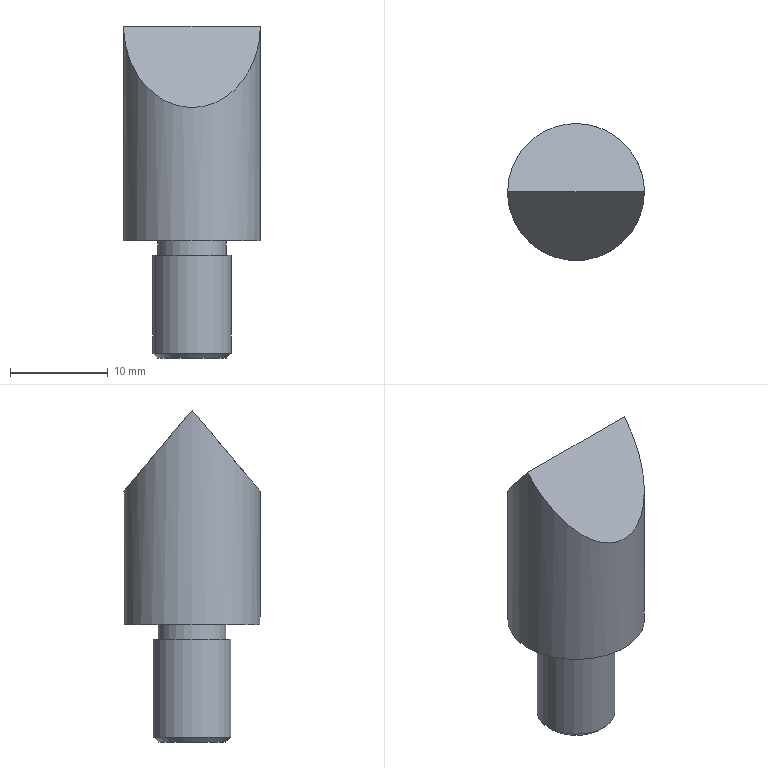Component | NX | SCRAP_CUTTER | 1 solid | 9 faces | box 14 x 14 x 34 mm | volume 3424 mm3 | plane 5 | cylinder 3 | cone 1 | commonest cylinder face diameters 8 x1 7 x1 14 x1
STEP:
#1=CARTESIAN_POINT('',(0.,0.,0.));
#2=DIRECTION('',(0.,0.,1.));
#3=DIRECTION('',(1.,0.,0.));
#4=AXIS2_PLACEMENT_3D('',#1,#2,#3);
#5=CARTESIAN_POINT('',(164.,0.,70.));
#6=VERTEX_POINT('',#5);
#7=CARTESIAN_POINT('',(150.,0.,70.));
#8=VERTEX_POINT('',#7);
#9=CARTESIAN_POINT('',(157.,0.,70.));
#10=DIRECTION('',(0.,0.766,-0.6428));
#11=DIRECTION('',(0.,-0.6428,-0.766));
#12=AXIS2_PLACEMENT_3D('',#9,#10,#11);
#13=ELLIPSE('',#12,10.89,7.);
#14=CARTESIAN_POINT('',(157.,0.,70.));
#15=DIRECTION('',(0.,-0.766,0.6428));
#16=DIRECTION('',(0.,0.6428,0.766));
#17=AXIS2_PLACEMENT_3D('',#14,#15,#16);
#18=PLANE('',#17);
#19=CARTESIAN_POINT('',(-10.89,0.));
#20=CARTESIAN_POINT('',(-10.89,12.124));
#21=CARTESIAN_POINT('',(5.445,6.062));
#22=CARTESIAN_POINT('',(21.78,0.));
#23=CARTESIAN_POINT('',(5.445,-6.062));
#24=CARTESIAN_POINT('',(-10.89,-12.124));
#25=CARTESIAN_POINT('',(-10.89,0.));
#26=(BOUNDED_CURVE()B_SPLINE_CURVE(2,(#19,#20,#21,#22,#23,#24,#25),.UNSPECIFIED.,.T.,.F.)B_SPLINE_CURVE_WITH_KNOTS((1,2,2,2,2,1),(-2.094,0.,2.094,4.189,6.283,8.378),.UNSPECIFIED.)CURVE()GEOMETRIC_REPRESENTATION_ITEM()RATIONAL_B_SPLINE_CURVE((1.,0.5,1.,0.5,1.,0.5,1.))REPRESENTATION_ITEM(''));
#27=(GEOMETRIC_REPRESENTATION_CONTEXT(2)PARAMETRIC_REPRESENTATION_CONTEXT()REPRESENTATION_CONTEXT('',''));
#28=DEFINITIONAL_REPRESENTATION('',(#26),#27);
#29=PCURVE('',#18,#28);
#30=CARTESIAN_POINT('',(157.,0.,70.));
#31=DIRECTION('',(0.,0.,-1.));
#32=DIRECTION('',(-1.,0.,0.));
#33=AXIS2_PLACEMENT_3D('',#30,#31,#32);
#34=CYLINDRICAL_SURFACE('',#33,7.);
#35=CARTESIAN_POINT('',(3.142,0.));
#36=CARTESIAN_POINT('',(3.189,0.3971));
#37=CARTESIAN_POINT('',(3.284,1.191));
#38=CARTESIAN_POINT('',(3.427,2.358));
#39=CARTESIAN_POINT('',(3.57,3.477));
#40=CARTESIAN_POINT('',(3.713,4.526));
#41=CARTESIAN_POINT('',(3.856,5.482));
#42=CARTESIAN_POINT('',(3.998,6.326));
#43=CARTESIAN_POINT('',(4.141,7.042));
#44=CARTESIAN_POINT('',(4.284,7.614));
#45=CARTESIAN_POINT('',(4.427,8.032));
#46=CARTESIAN_POINT('',(4.57,8.285));
#47=CARTESIAN_POINT('',(4.712,8.371));
#48=CARTESIAN_POINT('',(4.855,8.285));
#49=CARTESIAN_POINT('',(4.998,8.032));
#50=CARTESIAN_POINT('',(5.141,7.614));
#51=CARTESIAN_POINT('',(5.284,7.042));
#52=CARTESIAN_POINT('',(5.426,6.326));
#53=CARTESIAN_POINT('',(5.569,5.482));
#54=CARTESIAN_POINT('',(5.712,4.526));
#55=CARTESIAN_POINT('',(5.855,3.477));
#56=CARTESIAN_POINT('',(5.998,2.358));
#57=CARTESIAN_POINT('',(6.14,1.191));
#58=CARTESIAN_POINT('',(6.236,0.3971));
#59=CARTESIAN_POINT('',(6.283,0.));
#60=B_SPLINE_CURVE_WITH_KNOTS('',3,(#35,#36,#37,#38,#39,#40,#41,#42,#43,#44,#45,#46,#47,#48,#49,#50,#51,#52,#53,#54,#55,#56,#57,#58,#59),.UNSPECIFIED.,.F.,.F.,(4,1,1,1,1,1,1,1,1,1,1,1,1,1,1,1,1,1,1,1,1,1,4),(4.712,4.855,4.998,5.141,5.284,5.426,5.569,5.712,5.855,5.998,6.14,6.283,6.426,6.569,6.712,6.854,6.997,7.14,7.283,7.426,7.568,7.711,7.854),.QUASI_UNIFORM_KNOTS.);
#61=(GEOMETRIC_REPRESENTATION_CONTEXT(2)PARAMETRIC_REPRESENTATION_CONTEXT()REPRESENTATION_CONTEXT('',''));
#62=DEFINITIONAL_REPRESENTATION('',(#60),#61);
#63=PCURVE('',#34,#62);
#64=SURFACE_CURVE('',#13,(#29,#63),.PCURVE_S1.);
#65=EDGE_CURVE('',#6,#8,#64,.T.);
#66=ORIENTED_EDGE('',*,*,#65,.F.);
#67=CARTESIAN_POINT('',(164.,0.,70.));
#68=DIRECTION('',(-1.,0.,0.));
#69=VECTOR('',#68,1.);
#70=LINE('',#67,#69);
#71=CARTESIAN_POINT('',(0.,-7.));
#72=DIRECTION('',(0.,1.));
#73=VECTOR('',#72,1.);
#74=LINE('',#71,#73);
#75=(GEOMETRIC_REPRESENTATION_CONTEXT(2)PARAMETRIC_REPRESENTATION_CONTEXT()REPRESENTATION_CONTEXT('',''));
#76=DEFINITIONAL_REPRESENTATION('',(#74),#75);
#77=PCURVE('',#18,#76);
#78=CARTESIAN_POINT('',(157.,0.,70.));
#79=DIRECTION('',(0.,0.766,0.6428));
#80=DIRECTION('',(0.,-0.6428,0.766));
#81=AXIS2_PLACEMENT_3D('',#78,#79,#80);
#82=PLANE('',#81);
#83=CARTESIAN_POINT('',(0.,7.));
#84=DIRECTION('',(0.,-1.));
#85=VECTOR('',#84,1.);
#86=LINE('',#83,#85);
#87=(GEOMETRIC_REPRESENTATION_CONTEXT(2)PARAMETRIC_REPRESENTATION_CONTEXT()REPRESENTATION_CONTEXT('',''));
#88=DEFINITIONAL_REPRESENTATION('',(#86),#87);
#89=PCURVE('',#82,#88);
#90=SURFACE_CURVE('',#70,(#77,#89),.PCURVE_S1.);
#91=EDGE_CURVE('',#6,#8,#90,.T.);
#92=ORIENTED_EDGE('',*,*,#91,.T.);
#93=EDGE_LOOP('',(#66,#92));
#94=FACE_BOUND('',#93,.T.);
#95=ADVANCED_FACE('',(#94),#18,.T.);
#96=CARTESIAN_POINT('',(153.5,0.,36.));
#97=VERTEX_POINT('',#96);
#98=CARTESIAN_POINT('',(157.,0.,36.));
#99=DIRECTION('',(0.,0.,-1.));
#100=DIRECTION('',(-1.,0.,0.));
#101=AXIS2_PLACEMENT_3D('',#98,#99,#100);
#102=CIRCLE('',#101,3.5);
#103=CARTESIAN_POINT('',(157.,0.,36.));
#104=DIRECTION('',(0.,0.,-1.));
#105=DIRECTION('',(-1.,0.,0.));
#106=AXIS2_PLACEMENT_3D('',#103,#104,#105);
#107=PLANE('',#106);
#108=CARTESIAN_POINT('',(0.,0.));
#109=DIRECTION('',(1.,0.));
#110=AXIS2_PLACEMENT_2D('',#108,#109);
#111=CIRCLE('',#110,3.5);
#112=(GEOMETRIC_REPRESENTATION_CONTEXT(2)PARAMETRIC_REPRESENTATION_CONTEXT()REPRESENTATION_CONTEXT('',''));
#113=DEFINITIONAL_REPRESENTATION('',(#111),#112);
#114=PCURVE('',#107,#113);
#115=CARTESIAN_POINT('',(157.,0.,36.));
#116=DIRECTION('',(0.,0.,1.));
#117=DIRECTION('',(1.,0.,0.));
#118=AXIS2_PLACEMENT_3D('',#115,#116,#117);
#119=CONICAL_SURFACE('',#118,3.5,0.7854);
#120=CARTESIAN_POINT('',(9.425,0.));
#121=DIRECTION('',(-1.,0.));
#122=VECTOR('',#121,1.);
#123=LINE('',#120,#122);
#124=(GEOMETRIC_REPRESENTATION_CONTEXT(2)PARAMETRIC_REPRESENTATION_CONTEXT()REPRESENTATION_CONTEXT('',''));
#125=DEFINITIONAL_REPRESENTATION('',(#123),#124);
#126=PCURVE('',#119,#125);
#127=SURFACE_CURVE('',#102,(#114,#126),.PCURVE_S1.);
#128=EDGE_CURVE('',#97,#97,#127,.T.);
#129=ORIENTED_EDGE('',*,*,#128,.T.);
#130=EDGE_LOOP('',(#129));
#131=FACE_BOUND('',#130,.T.);
#132=ADVANCED_FACE('',(#131),#107,.T.);
#133=CARTESIAN_POINT('',(153.,0.,36.5));
#134=VERTEX_POINT('',#133);
#135=CARTESIAN_POINT('',(157.,0.,36.5));
#136=DIRECTION('',(0.,0.,-1.));
#137=DIRECTION('',(-1.,0.,0.));
#138=AXIS2_PLACEMENT_3D('',#135,#136,#137);
#139=CIRCLE('',#138,4.);
#140=CARTESIAN_POINT('',(9.425,0.5));
#141=DIRECTION('',(-1.,0.));
#142=VECTOR('',#141,1.);
#143=LINE('',#140,#142);
#144=(GEOMETRIC_REPRESENTATION_CONTEXT(2)PARAMETRIC_REPRESENTATION_CONTEXT()REPRESENTATION_CONTEXT('',''));
#145=DEFINITIONAL_REPRESENTATION('',(#143),#144);
#146=PCURVE('',#119,#145);
#147=CARTESIAN_POINT('',(157.,0.,70.));
#148=DIRECTION('',(0.,0.,-1.));
#149=DIRECTION('',(-1.,0.,0.));
#150=AXIS2_PLACEMENT_3D('',#147,#148,#149);
#151=CYLINDRICAL_SURFACE('',#150,4.);
#152=CARTESIAN_POINT('',(0.,33.5));
#153=DIRECTION('',(1.,0.));
#154=VECTOR('',#153,1.);
#155=LINE('',#152,#154);
#156=(GEOMETRIC_REPRESENTATION_CONTEXT(2)PARAMETRIC_REPRESENTATION_CONTEXT()REPRESENTATION_CONTEXT('',''));
#157=DEFINITIONAL_REPRESENTATION('',(#155),#156);
#158=PCURVE('',#151,#157);
#159=SURFACE_CURVE('',#139,(#146,#158),.PCURVE_S1.);
#160=EDGE_CURVE('',#134,#134,#159,.T.);
#161=ORIENTED_EDGE('',*,*,#160,.T.);
#162=CARTESIAN_POINT('',(153.5,0.,36.));
#163=CARTESIAN_POINT('',(153.,0.,36.5));
#164=B_SPLINE_CURVE_WITH_KNOTS('',1,(#162,#163),.UNSPECIFIED.,.F.,.F.,(2,2),(0.,0.7071),.PIECEWISE_BEZIER_KNOTS.);
#165=CARTESIAN_POINT('',(3.142,0.));
#166=DIRECTION('',(0.,1.));
#167=VECTOR('',#166,1.);
#168=LINE('',#165,#167);
#169=(GEOMETRIC_REPRESENTATION_CONTEXT(2)PARAMETRIC_REPRESENTATION_CONTEXT()REPRESENTATION_CONTEXT('',''));
#170=DEFINITIONAL_REPRESENTATION('',(#168),#169);
#171=PCURVE('',#119,#170);
#172=CARTESIAN_POINT('',(9.425,0.));
#173=DIRECTION('',(0.,1.));
#174=VECTOR('',#173,1.);
#175=LINE('',#172,#174);
#176=(GEOMETRIC_REPRESENTATION_CONTEXT(2)PARAMETRIC_REPRESENTATION_CONTEXT()REPRESENTATION_CONTEXT('',''));
#177=DEFINITIONAL_REPRESENTATION('',(#175),#176);
#178=PCURVE('',#119,#177);
#179=SEAM_CURVE('',#164,(#171,#178),.PCURVE_S1.);
#180=EDGE_CURVE('',#97,#134,#179,.T.);
#181=ORIENTED_EDGE('',*,*,#180,.F.);
#182=ORIENTED_EDGE('',*,*,#128,.F.);
#183=ORIENTED_EDGE('',*,*,#180,.T.);
#184=EDGE_LOOP('',(#161,#181,#182,#183));
#185=FACE_BOUND('',#184,.T.);
#186=ADVANCED_FACE('',(#185),#119,.T.);
#187=CARTESIAN_POINT('',(153.,0.,46.5));
#188=VERTEX_POINT('',#187);
#189=CARTESIAN_POINT('',(157.,0.,46.5));
#190=DIRECTION('',(0.,0.,-1.));
#191=DIRECTION('',(-1.,0.,0.));
#192=AXIS2_PLACEMENT_3D('',#189,#190,#191);
#193=CIRCLE('',#192,4.);
#194=CARTESIAN_POINT('',(0.,23.5));
#195=DIRECTION('',(1.,0.));
#196=VECTOR('',#195,1.);
#197=LINE('',#194,#196);
#198=(GEOMETRIC_REPRESENTATION_CONTEXT(2)PARAMETRIC_REPRESENTATION_CONTEXT()REPRESENTATION_CONTEXT('',''));
#199=DEFINITIONAL_REPRESENTATION('',(#197),#198);
#200=PCURVE('',#151,#199);
#201=CARTESIAN_POINT('',(161.,0.,46.5));
#202=DIRECTION('',(0.,0.,1.));
#203=DIRECTION('',(1.,0.,0.));
#204=AXIS2_PLACEMENT_3D('',#201,#202,#203);
#205=PLANE('',#204);
#206=CARTESIAN_POINT('',(-8.,0.));
#207=CARTESIAN_POINT('',(-8.,6.928));
#208=CARTESIAN_POINT('',(-2.,3.464));
#209=CARTESIAN_POINT('',(4.,0.));
#210=CARTESIAN_POINT('',(-2.,-3.464));
#211=CARTESIAN_POINT('',(-8.,-6.928));
#212=CARTESIAN_POINT('',(-8.,0.));
#213=(BOUNDED_CURVE()B_SPLINE_CURVE(2,(#206,#207,#208,#209,#210,#211,#212),.UNSPECIFIED.,.T.,.F.)B_SPLINE_CURVE_WITH_KNOTS((1,2,2,2,2,1),(-2.094,0.,2.094,4.189,6.283,8.378),.UNSPECIFIED.)CURVE()GEOMETRIC_REPRESENTATION_ITEM()RATIONAL_B_SPLINE_CURVE((1.,0.5,1.,0.5,1.,0.5,1.))REPRESENTATION_ITEM(''));
#214=(GEOMETRIC_REPRESENTATION_CONTEXT(2)PARAMETRIC_REPRESENTATION_CONTEXT()REPRESENTATION_CONTEXT('',''));
#215=DEFINITIONAL_REPRESENTATION('',(#213),#214);
#216=PCURVE('',#205,#215);
#217=SURFACE_CURVE('',#193,(#200,#216),.PCURVE_S1.);
#218=EDGE_CURVE('',#188,#188,#217,.T.);
#219=ORIENTED_EDGE('',*,*,#218,.T.);
#220=CARTESIAN_POINT('',(153.,0.,46.5));
#221=CARTESIAN_POINT('',(153.,0.,36.5));
#222=B_SPLINE_CURVE_WITH_KNOTS('',1,(#220,#221),.UNSPECIFIED.,.F.,.F.,(2,2),(23.5,33.5),.PIECEWISE_BEZIER_KNOTS.);
#223=CARTESIAN_POINT('',(6.283,0.));
#224=DIRECTION('',(0.,1.));
#225=VECTOR('',#224,1.);
#226=LINE('',#223,#225);
#227=(GEOMETRIC_REPRESENTATION_CONTEXT(2)PARAMETRIC_REPRESENTATION_CONTEXT()REPRESENTATION_CONTEXT('',''));
#228=DEFINITIONAL_REPRESENTATION('',(#226),#227);
#229=PCURVE('',#151,#228);
#230=CARTESIAN_POINT('',(0.,0.));
#231=DIRECTION('',(0.,1.));
#232=VECTOR('',#231,1.);
#233=LINE('',#230,#232);
#234=(GEOMETRIC_REPRESENTATION_CONTEXT(2)PARAMETRIC_REPRESENTATION_CONTEXT()REPRESENTATION_CONTEXT('',''));
#235=DEFINITIONAL_REPRESENTATION('',(#233),#234);
#236=PCURVE('',#151,#235);
#237=SEAM_CURVE('',#222,(#229,#236),.PCURVE_S1.);
#238=EDGE_CURVE('',#188,#134,#237,.T.);
#239=ORIENTED_EDGE('',*,*,#238,.T.);
#240=ORIENTED_EDGE('',*,*,#160,.F.);
#241=ORIENTED_EDGE('',*,*,#238,.F.);
#242=EDGE_LOOP('',(#219,#239,#240,#241));
#243=FACE_BOUND('',#242,.T.);
#244=ADVANCED_FACE('',(#243),#151,.T.);
#245=CARTESIAN_POINT('',(153.5,0.,46.5));
#246=VERTEX_POINT('',#245);
#247=CARTESIAN_POINT('',(157.,0.,46.5));
#248=DIRECTION('',(0.,0.,-1.));
#249=DIRECTION('',(-1.,0.,0.));
#250=AXIS2_PLACEMENT_3D('',#247,#248,#249);
#251=CIRCLE('',#250,3.5);
#252=CARTESIAN_POINT('',(-7.5,0.));
#253=CARTESIAN_POINT('',(-7.5,6.062));
#254=CARTESIAN_POINT('',(-2.25,3.031));
#255=CARTESIAN_POINT('',(3.,0.));
#256=CARTESIAN_POINT('',(-2.25,-3.031));
#257=CARTESIAN_POINT('',(-7.5,-6.062));
#258=CARTESIAN_POINT('',(-7.5,0.));
#259=(BOUNDED_CURVE()B_SPLINE_CURVE(2,(#252,#253,#254,#255,#256,#257,#258),.UNSPECIFIED.,.T.,.F.)B_SPLINE_CURVE_WITH_KNOTS((1,2,2,2,2,1),(-2.094,0.,2.094,4.189,6.283,8.378),.UNSPECIFIED.)CURVE()GEOMETRIC_REPRESENTATION_ITEM()RATIONAL_B_SPLINE_CURVE((1.,0.5,1.,0.5,1.,0.5,1.))REPRESENTATION_ITEM(''));
#260=(GEOMETRIC_REPRESENTATION_CONTEXT(2)PARAMETRIC_REPRESENTATION_CONTEXT()REPRESENTATION_CONTEXT('',''));
#261=DEFINITIONAL_REPRESENTATION('',(#259),#260);
#262=PCURVE('',#205,#261);
#263=CARTESIAN_POINT('',(157.,0.,70.));
#264=DIRECTION('',(0.,0.,-1.));
#265=DIRECTION('',(-1.,0.,0.));
#266=AXIS2_PLACEMENT_3D('',#263,#264,#265);
#267=CYLINDRICAL_SURFACE('',#266,3.5);
#268=CARTESIAN_POINT('',(0.,23.5));
#269=DIRECTION('',(1.,0.));
#270=VECTOR('',#269,1.);
#271=LINE('',#268,#270);
#272=(GEOMETRIC_REPRESENTATION_CONTEXT(2)PARAMETRIC_REPRESENTATION_CONTEXT()REPRESENTATION_CONTEXT('',''));
#273=DEFINITIONAL_REPRESENTATION('',(#271),#272);
#274=PCURVE('',#267,#273);
#275=SURFACE_CURVE('',#251,(#262,#274),.PCURVE_S1.);
#276=EDGE_CURVE('',#246,#246,#275,.T.);
#277=ORIENTED_EDGE('',*,*,#276,.T.);
#278=EDGE_LOOP('',(#277));
#279=FACE_BOUND('',#278,.T.);
#280=ORIENTED_EDGE('',*,*,#218,.F.);
#281=EDGE_LOOP('',(#280));
#282=FACE_BOUND('',#281,.T.);
#283=ADVANCED_FACE('',(#279,#282),#205,.T.);
#284=CARTESIAN_POINT('',(153.5,0.,48.));
#285=VERTEX_POINT('',#284);
#286=CARTESIAN_POINT('',(157.,0.,48.));
#287=DIRECTION('',(0.,0.,-1.));
#288=DIRECTION('',(-1.,0.,0.));
#289=AXIS2_PLACEMENT_3D('',#286,#287,#288);
#290=CIRCLE('',#289,3.5);
#291=CARTESIAN_POINT('',(0.,22.));
#292=DIRECTION('',(1.,0.));
#293=VECTOR('',#292,1.);
#294=LINE('',#291,#293);
#295=(GEOMETRIC_REPRESENTATION_CONTEXT(2)PARAMETRIC_REPRESENTATION_CONTEXT()REPRESENTATION_CONTEXT('',''));
#296=DEFINITIONAL_REPRESENTATION('',(#294),#295);
#297=PCURVE('',#267,#296);
#298=CARTESIAN_POINT('',(160.5,0.,48.));
#299=DIRECTION('',(0.,0.,-1.));
#300=DIRECTION('',(-1.,0.,0.));
#301=AXIS2_PLACEMENT_3D('',#298,#299,#300);
#302=PLANE('',#301);
#303=CARTESIAN_POINT('',(3.5,0.));
#304=DIRECTION('',(1.,0.));
#305=AXIS2_PLACEMENT_2D('',#303,#304);
#306=CIRCLE('',#305,3.5);
#307=(GEOMETRIC_REPRESENTATION_CONTEXT(2)PARAMETRIC_REPRESENTATION_CONTEXT()REPRESENTATION_CONTEXT('',''));
#308=DEFINITIONAL_REPRESENTATION('',(#306),#307);
#309=PCURVE('',#302,#308);
#310=SURFACE_CURVE('',#290,(#297,#309),.PCURVE_S1.);
#311=EDGE_CURVE('',#285,#285,#310,.T.);
#312=ORIENTED_EDGE('',*,*,#311,.T.);
#313=CARTESIAN_POINT('',(153.5,0.,48.));
#314=CARTESIAN_POINT('',(153.5,0.,46.5));
#315=B_SPLINE_CURVE_WITH_KNOTS('',1,(#313,#314),.UNSPECIFIED.,.F.,.F.,(2,2),(22.,23.5),.PIECEWISE_BEZIER_KNOTS.);
#316=CARTESIAN_POINT('',(6.283,0.));
#317=DIRECTION('',(0.,1.));
#318=VECTOR('',#317,1.);
#319=LINE('',#316,#318);
#320=(GEOMETRIC_REPRESENTATION_CONTEXT(2)PARAMETRIC_REPRESENTATION_CONTEXT()REPRESENTATION_CONTEXT('',''));
#321=DEFINITIONAL_REPRESENTATION('',(#319),#320);
#322=PCURVE('',#267,#321);
#323=CARTESIAN_POINT('',(0.,0.));
#324=DIRECTION('',(0.,1.));
#325=VECTOR('',#324,1.);
#326=LINE('',#323,#325);
#327=(GEOMETRIC_REPRESENTATION_CONTEXT(2)PARAMETRIC_REPRESENTATION_CONTEXT()REPRESENTATION_CONTEXT('',''));
#328=DEFINITIONAL_REPRESENTATION('',(#326),#327);
#329=PCURVE('',#267,#328);
#330=SEAM_CURVE('',#315,(#322,#329),.PCURVE_S1.);
#331=EDGE_CURVE('',#285,#246,#330,.T.);
#332=ORIENTED_EDGE('',*,*,#331,.T.);
#333=ORIENTED_EDGE('',*,*,#276,.F.);
#334=ORIENTED_EDGE('',*,*,#331,.F.);
#335=EDGE_LOOP('',(#312,#332,#333,#334));
#336=FACE_BOUND('',#335,.T.);
#337=ADVANCED_FACE('',(#336),#267,.T.);
#338=CARTESIAN_POINT('',(157.,0.,70.));
#339=DIRECTION('',(0.,-0.766,-0.6428));
#340=DIRECTION('',(0.,0.6428,-0.766));
#341=AXIS2_PLACEMENT_3D('',#338,#339,#340);
#342=ELLIPSE('',#341,10.89,7.);
#343=CARTESIAN_POINT('',(-10.89,0.));
#344=CARTESIAN_POINT('',(-10.89,12.124));
#345=CARTESIAN_POINT('',(5.445,6.062));
#346=CARTESIAN_POINT('',(21.78,0.));
#347=CARTESIAN_POINT('',(5.445,-6.062));
#348=CARTESIAN_POINT('',(-10.89,-12.124));
#349=CARTESIAN_POINT('',(-10.89,0.));
#350=(BOUNDED_CURVE()B_SPLINE_CURVE(2,(#343,#344,#345,#346,#347,#348,#349),.UNSPECIFIED.,.T.,.F.)B_SPLINE_CURVE_WITH_KNOTS((1,2,2,2,2,1),(-2.094,0.,2.094,4.189,6.283,8.378),.UNSPECIFIED.)CURVE()GEOMETRIC_REPRESENTATION_ITEM()RATIONAL_B_SPLINE_CURVE((1.,0.5,1.,0.5,1.,0.5,1.))REPRESENTATION_ITEM(''));
#351=(GEOMETRIC_REPRESENTATION_CONTEXT(2)PARAMETRIC_REPRESENTATION_CONTEXT()REPRESENTATION_CONTEXT('',''));
#352=DEFINITIONAL_REPRESENTATION('',(#350),#351);
#353=PCURVE('',#82,#352);
#354=CARTESIAN_POINT('',(0.,0.));
#355=CARTESIAN_POINT('',(0.0476,0.3971));
#356=CARTESIAN_POINT('',(0.1428,1.191));
#357=CARTESIAN_POINT('',(0.2856,2.358));
#358=CARTESIAN_POINT('',(0.4284,3.477));
#359=CARTESIAN_POINT('',(0.5712,4.526));
#360=CARTESIAN_POINT('',(0.714,5.482));
#361=CARTESIAN_POINT('',(0.8568,6.326));
#362=CARTESIAN_POINT('',(0.9996,7.042));
#363=CARTESIAN_POINT('',(1.142,7.614));
#364=CARTESIAN_POINT('',(1.285,8.032));
#365=CARTESIAN_POINT('',(1.428,8.285));
#366=CARTESIAN_POINT('',(1.571,8.371));
#367=CARTESIAN_POINT('',(1.714,8.285));
#368=CARTESIAN_POINT('',(1.856,8.032));
#369=CARTESIAN_POINT('',(1.999,7.614));
#370=CARTESIAN_POINT('',(2.142,7.042));
#371=CARTESIAN_POINT('',(2.285,6.326));
#372=CARTESIAN_POINT('',(2.428,5.482));
#373=CARTESIAN_POINT('',(2.57,4.526));
#374=CARTESIAN_POINT('',(2.713,3.477));
#375=CARTESIAN_POINT('',(2.856,2.358));
#376=CARTESIAN_POINT('',(2.999,1.191));
#377=CARTESIAN_POINT('',(3.094,0.3971));
#378=CARTESIAN_POINT('',(3.142,0.));
#379=B_SPLINE_CURVE_WITH_KNOTS('',3,(#354,#355,#356,#357,#358,#359,#360,#361,#362,#363,#364,#365,#366,#367,#368,#369,#370,#371,#372,#373,#374,#375,#376,#377,#378),.UNSPECIFIED.,.F.,.F.,(4,1,1,1,1,1,1,1,1,1,1,1,1,1,1,1,1,1,1,1,1,1,4),(4.712,4.855,4.998,5.141,5.284,5.426,5.569,5.712,5.855,5.998,6.14,6.283,6.426,6.569,6.712,6.854,6.997,7.14,7.283,7.426,7.568,7.711,7.854),.QUASI_UNIFORM_KNOTS.);
#380=(GEOMETRIC_REPRESENTATION_CONTEXT(2)PARAMETRIC_REPRESENTATION_CONTEXT()REPRESENTATION_CONTEXT('',''));
#381=DEFINITIONAL_REPRESENTATION('',(#379),#380);
#382=PCURVE('',#34,#381);
#383=SURFACE_CURVE('',#342,(#353,#382),.PCURVE_S1.);
#384=EDGE_CURVE('',#8,#6,#383,.T.);
#385=ORIENTED_EDGE('',*,*,#384,.F.);
#386=ORIENTED_EDGE('',*,*,#91,.F.);
#387=EDGE_LOOP('',(#385,#386));
#388=FACE_BOUND('',#387,.T.);
#389=ADVANCED_FACE('',(#388),#82,.T.);
#390=CARTESIAN_POINT('',(150.,0.,48.));
#391=VERTEX_POINT('',#390);
#392=CARTESIAN_POINT('',(157.,0.,48.));
#393=DIRECTION('',(0.,0.,-1.));
#394=DIRECTION('',(-1.,0.,0.));
#395=AXIS2_PLACEMENT_3D('',#392,#393,#394);
#396=CIRCLE('',#395,7.);
#397=CARTESIAN_POINT('',(3.5,0.));
#398=DIRECTION('',(1.,0.));
#399=AXIS2_PLACEMENT_2D('',#397,#398);
#400=CIRCLE('',#399,7.);
#401=(GEOMETRIC_REPRESENTATION_CONTEXT(2)PARAMETRIC_REPRESENTATION_CONTEXT()REPRESENTATION_CONTEXT('',''));
#402=DEFINITIONAL_REPRESENTATION('',(#400),#401);
#403=PCURVE('',#302,#402);
#404=CARTESIAN_POINT('',(0.,22.));
#405=DIRECTION('',(1.,0.));
#406=VECTOR('',#405,1.);
#407=LINE('',#404,#406);
#408=(GEOMETRIC_REPRESENTATION_CONTEXT(2)PARAMETRIC_REPRESENTATION_CONTEXT()REPRESENTATION_CONTEXT('',''));
#409=DEFINITIONAL_REPRESENTATION('',(#407),#408);
#410=PCURVE('',#34,#409);
#411=SURFACE_CURVE('',#396,(#403,#410),.PCURVE_S1.);
#412=EDGE_CURVE('',#391,#391,#411,.T.);
#413=ORIENTED_EDGE('',*,*,#412,.T.);
#414=EDGE_LOOP('',(#413));
#415=FACE_BOUND('',#414,.T.);
#416=ORIENTED_EDGE('',*,*,#311,.F.);
#417=EDGE_LOOP('',(#416));
#418=FACE_BOUND('',#417,.T.);
#419=ADVANCED_FACE('',(#415,#418),#302,.T.);
#420=ORIENTED_EDGE('',*,*,#412,.F.);
#421=CARTESIAN_POINT('',(150.,-0.,70.));
#422=CARTESIAN_POINT('',(150.,-0.,48.));
#423=B_SPLINE_CURVE_WITH_KNOTS('',1,(#421,#422),.UNSPECIFIED.,.F.,.F.,(2,2),(0.,22.),.PIECEWISE_BEZIER_KNOTS.);
#424=CARTESIAN_POINT('',(0.,0.));
#425=DIRECTION('',(0.,1.));
#426=VECTOR('',#425,1.);
#427=LINE('',#424,#426);
#428=(GEOMETRIC_REPRESENTATION_CONTEXT(2)PARAMETRIC_REPRESENTATION_CONTEXT()REPRESENTATION_CONTEXT('',''));
#429=DEFINITIONAL_REPRESENTATION('',(#427),#428);
#430=PCURVE('',#34,#429);
#431=CARTESIAN_POINT('',(6.283,0.));
#432=DIRECTION('',(0.,1.));
#433=VECTOR('',#432,1.);
#434=LINE('',#431,#433);
#435=(GEOMETRIC_REPRESENTATION_CONTEXT(2)PARAMETRIC_REPRESENTATION_CONTEXT()REPRESENTATION_CONTEXT('',''));
#436=DEFINITIONAL_REPRESENTATION('',(#434),#435);
#437=PCURVE('',#34,#436);
#438=SEAM_CURVE('',#423,(#430,#437),.PCURVE_S1.);
#439=EDGE_CURVE('',#8,#391,#438,.T.);
#440=ORIENTED_EDGE('',*,*,#439,.F.);
#441=ORIENTED_EDGE('',*,*,#384,.T.);
#442=ORIENTED_EDGE('',*,*,#65,.T.);
#443=ORIENTED_EDGE('',*,*,#439,.T.);
#444=EDGE_LOOP('',(#420,#440,#441,#442,#443));
#445=FACE_BOUND('',#444,.T.);
#446=ADVANCED_FACE('',(#445),#34,.T.);
#447=CLOSED_SHELL('',(#95,#132,#186,#244,#283,#337,#389,#419,#446));
#448=MANIFOLD_SOLID_BREP('',#447);
#449=(LENGTH_UNIT()NAMED_UNIT(*)SI_UNIT(.MILLI.,.METRE.));
#450=UNCERTAINTY_MEASURE_WITH_UNIT(LENGTH_MEASURE(0.000005),#449,'','');
#451=(NAMED_UNIT(*)PLANE_ANGLE_UNIT()SI_UNIT($,.RADIAN.));
#452=(NAMED_UNIT(*)SI_UNIT($,.STERADIAN.)SOLID_ANGLE_UNIT());
#453=(GEOMETRIC_REPRESENTATION_CONTEXT(3)GLOBAL_UNCERTAINTY_ASSIGNED_CONTEXT((#450))GLOBAL_UNIT_ASSIGNED_CONTEXT((#449,#451,#452))REPRESENTATION_CONTEXT('',''));
#454=ADVANCED_BREP_SHAPE_REPRESENTATION('',(#4,#448),#453);